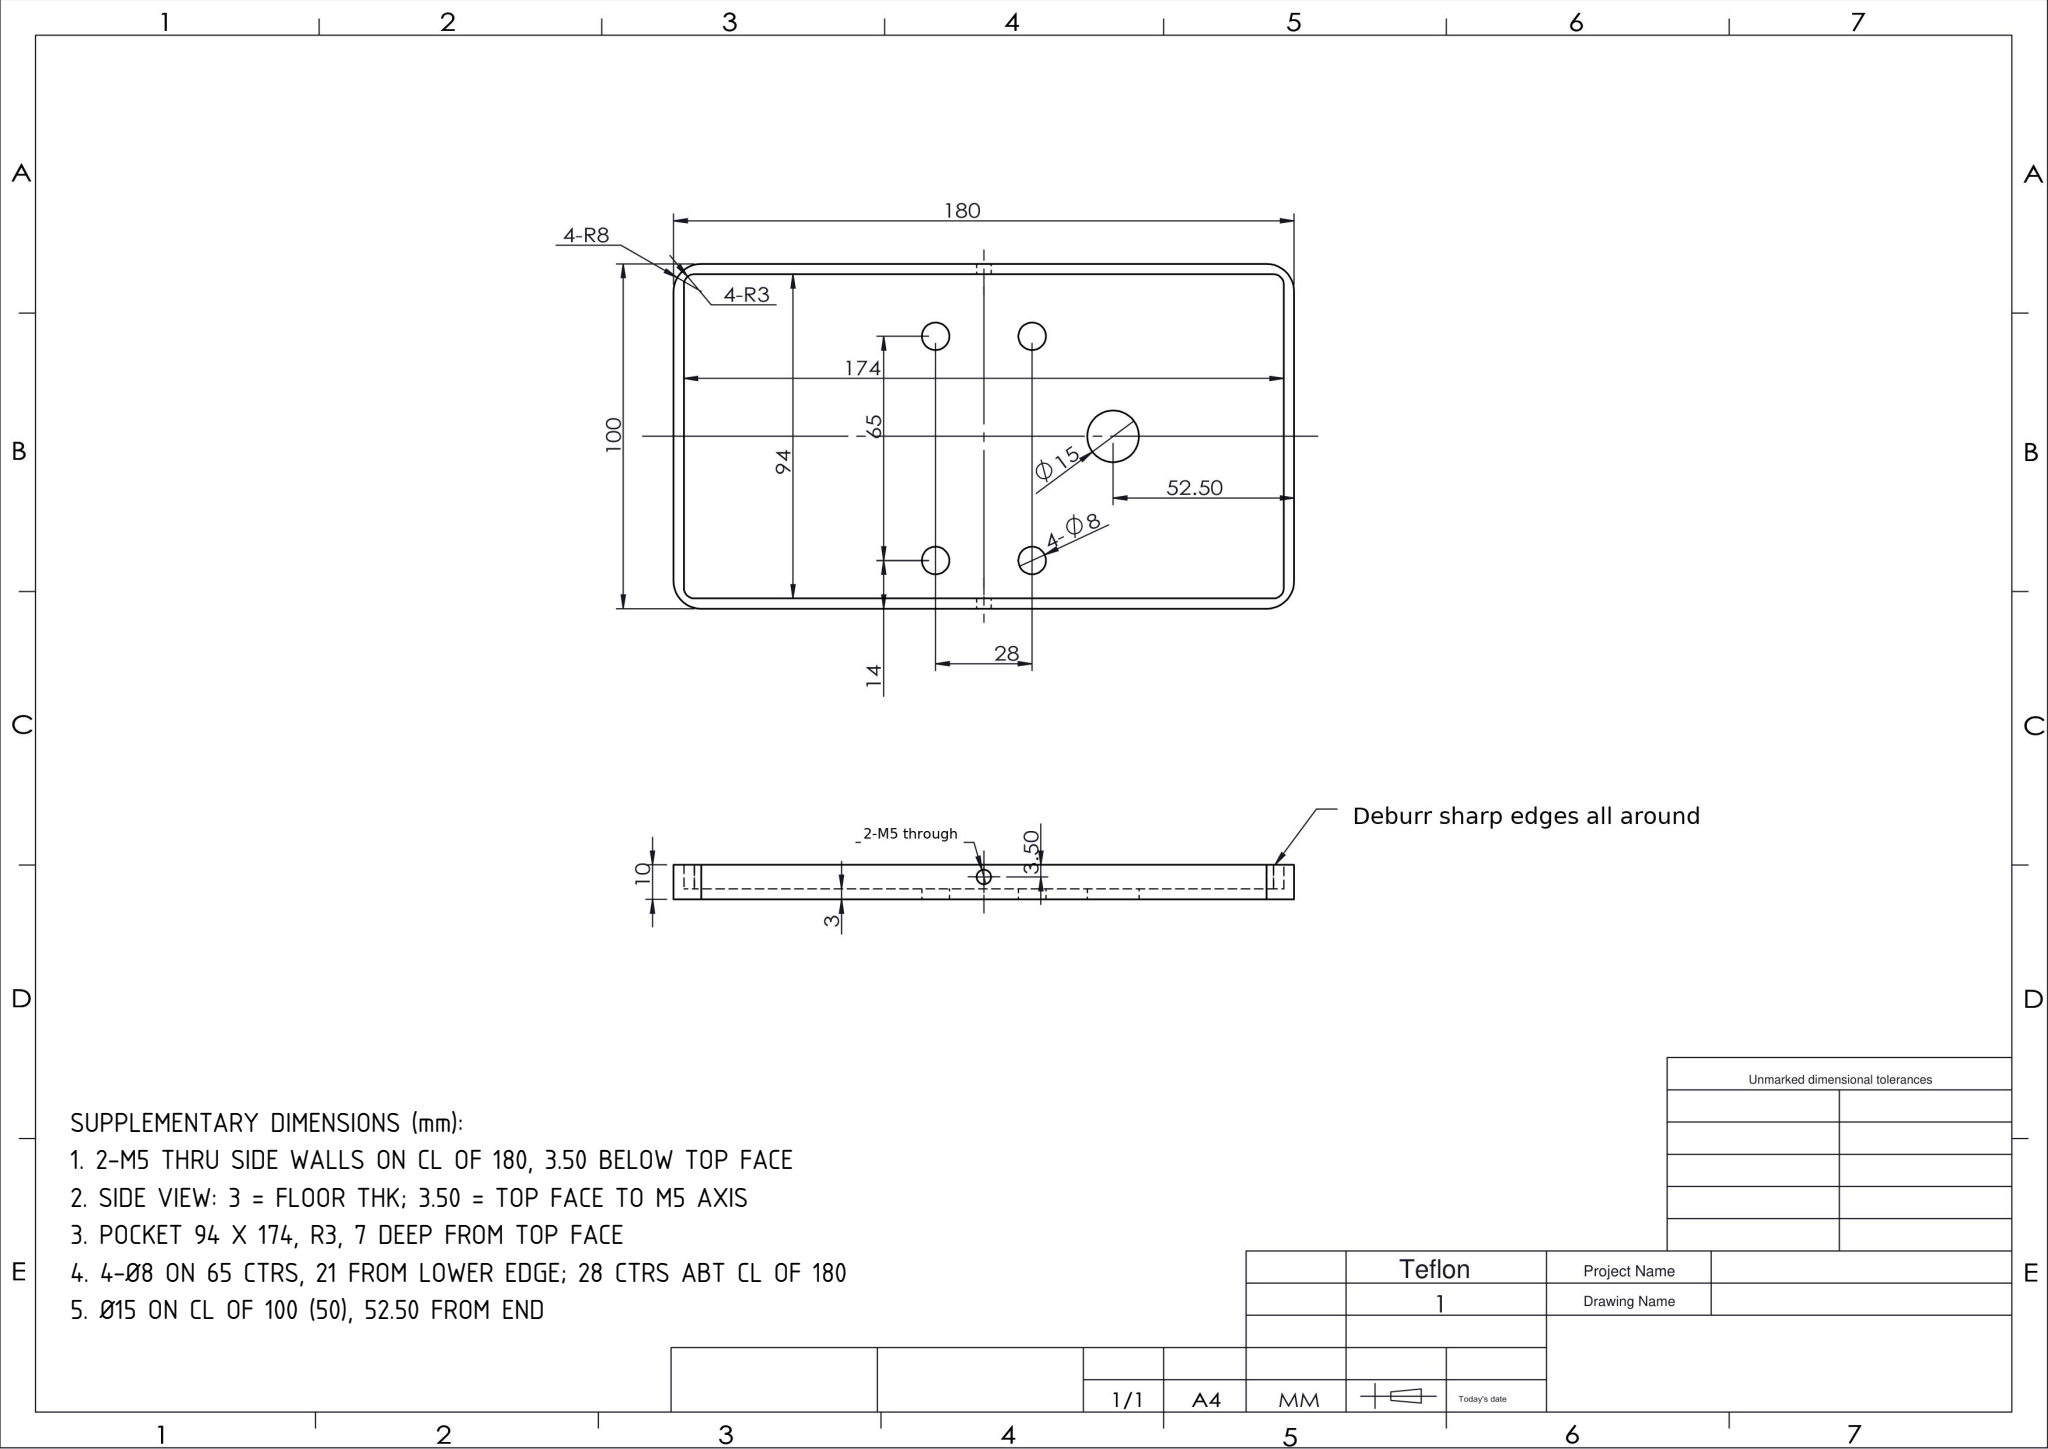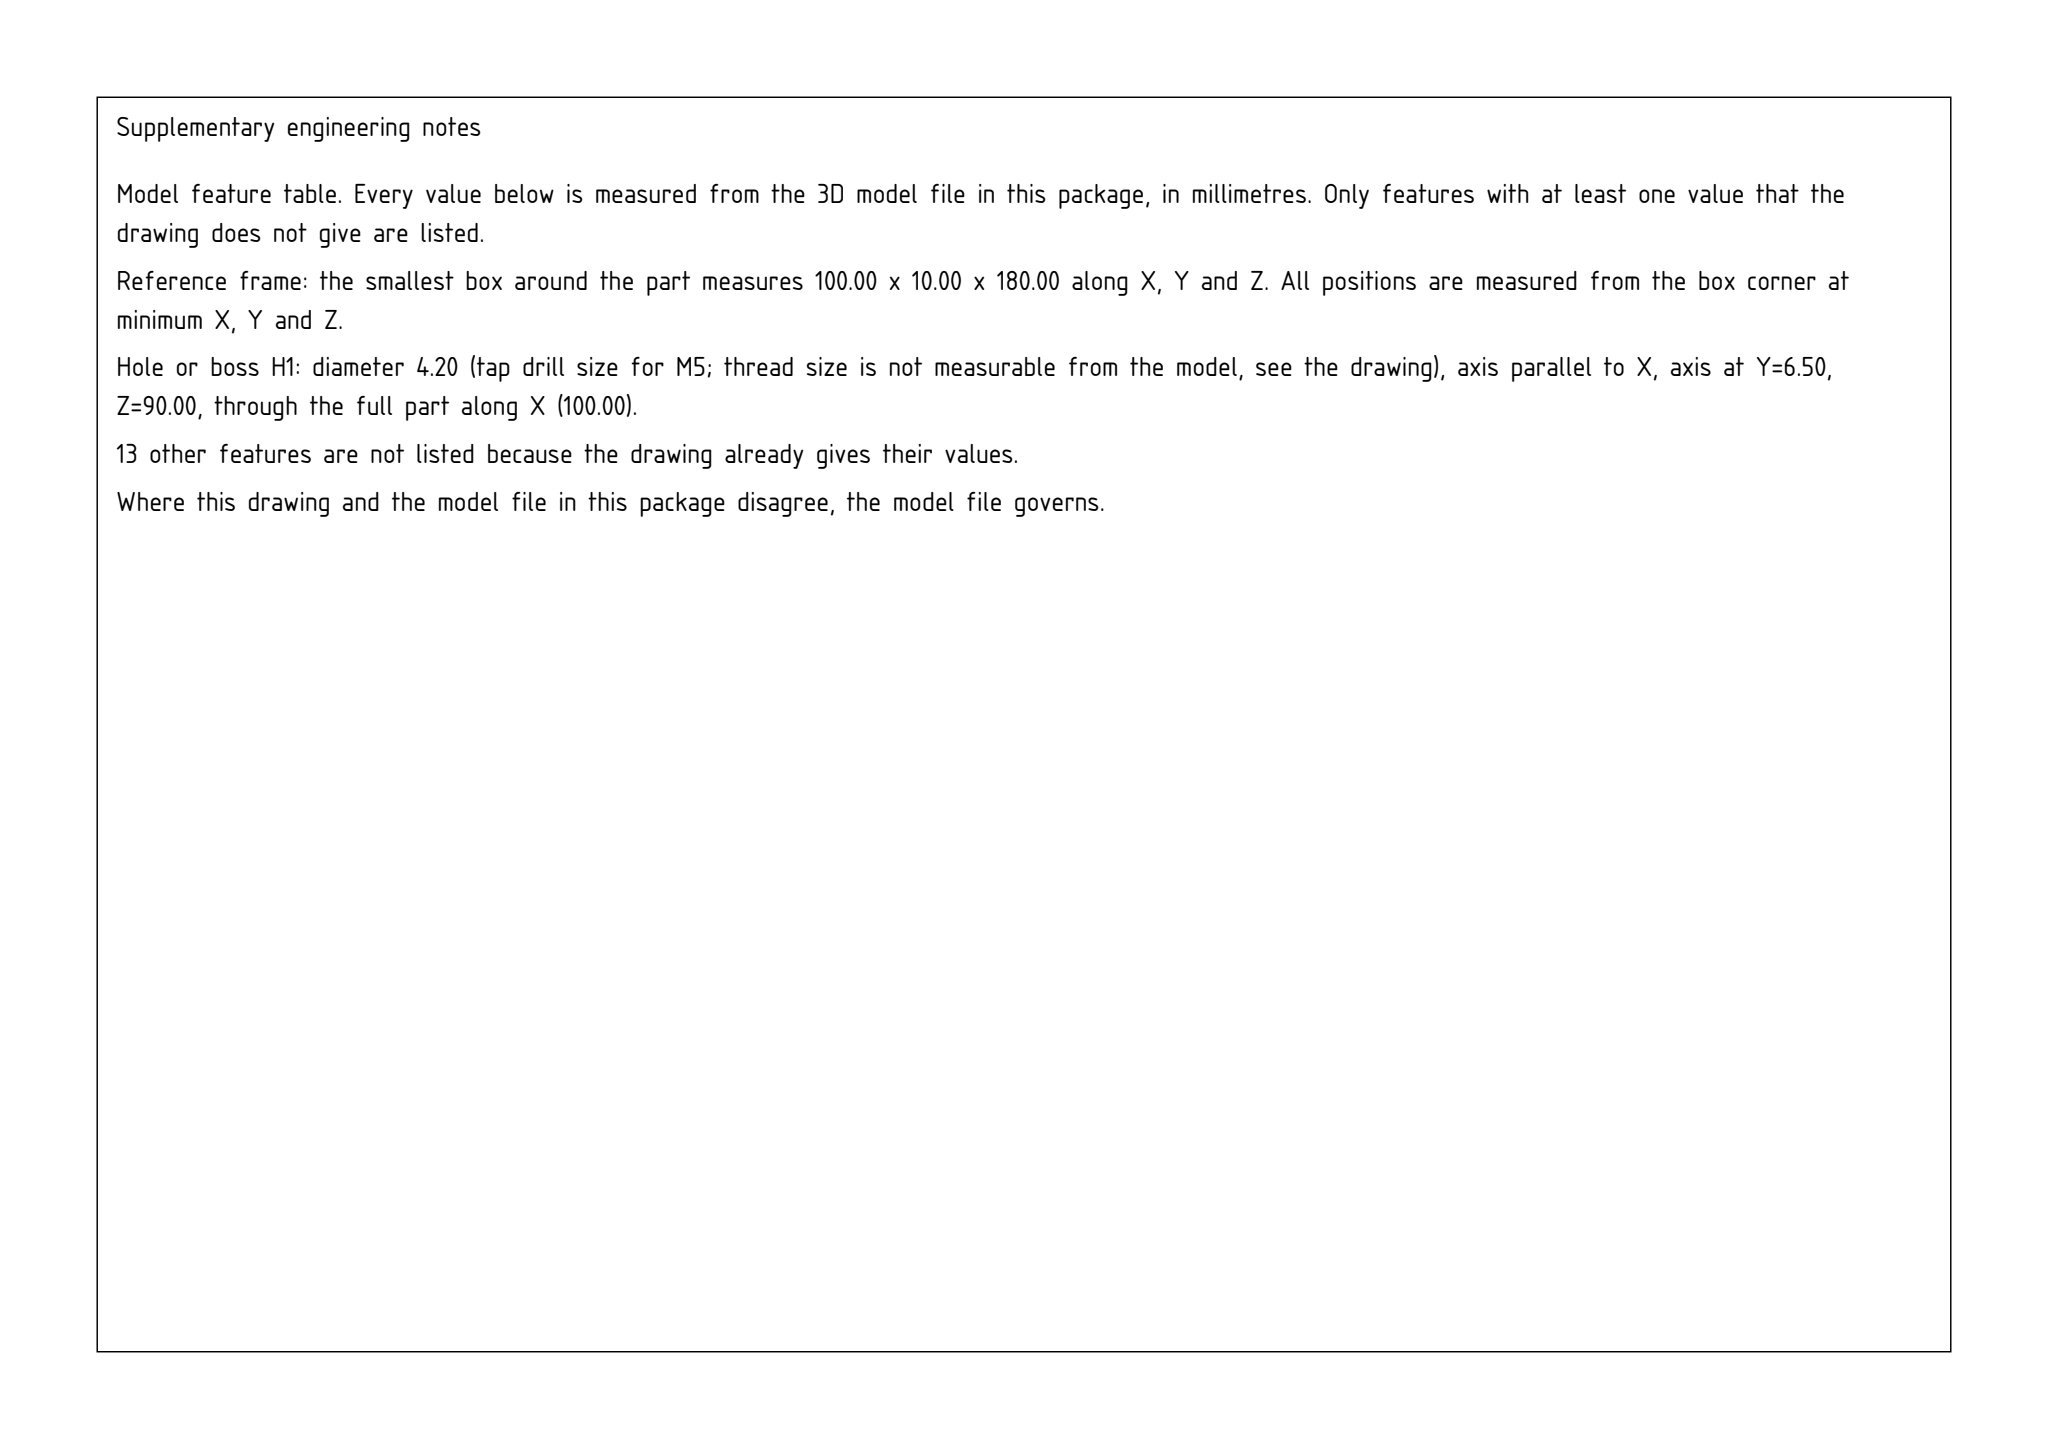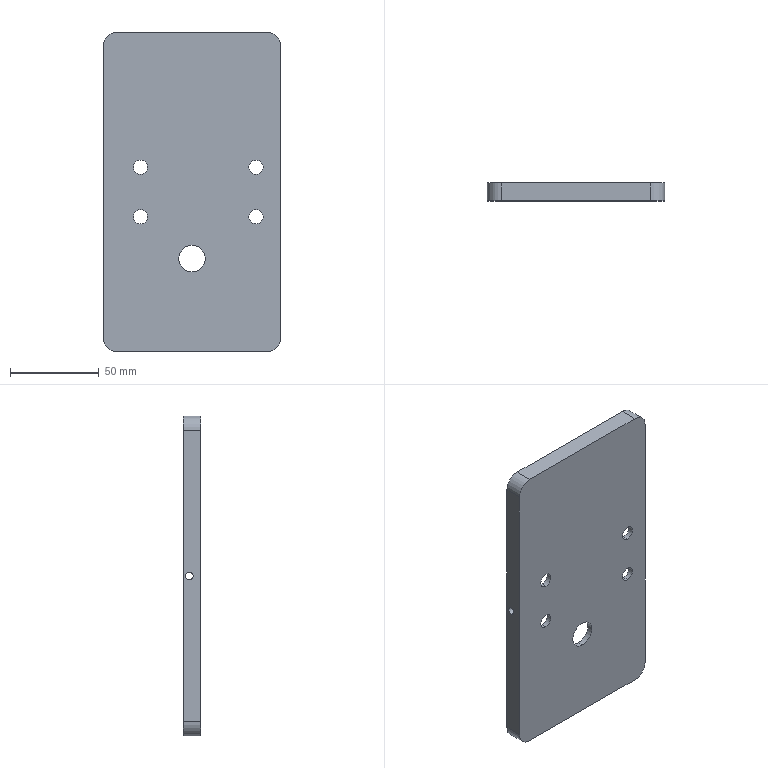Part | SolidWorks | mm | 1 solid | 33 faces | box 100 x 10 x 180 mm | volume 63796 mm3 | cylinder 22 | plane 11 | commonest cylinder face diameters 8 x8 4.2 x4 6 x4 16 x4 15 x2
build123d program:
from build123d import *

# Parameters (mm, degrees)
SKETCH1_W           = 100
SKETCH1_H           = 10
BOSS_EXTRUDE1_DEPTH = 180
SHELL1_T            = -3
M5_TAPPED_HOLE1_D   = 4.2
SKETCH5_R           = 7.5
CUT_EXTRUDE1_DEPTH  = 207.032
FILLET1_R           = 3
FILLET2_R           = 8
SKETCH6_R           = 4
CUT_EXTRUDE2_DEPTH  = 207.032


with BuildPart() as part:
    # Sketch1 → Boss-Extrude1 (new body)
    with BuildSketch(Plane.XY):
        with Locations((50, 5)):
            Rectangle(SKETCH1_W, SKETCH1_H)
    extrude(amount=BOSS_EXTRUDE1_DEPTH)

    # Shell1
    shell1_openings = [part.faces().sort_by_distance(p)[0] for p in [
        (50, 10, 90),
    ]]
    offset(amount=SHELL1_T, openings=shell1_openings, kind=Kind.INTERSECTION)

    # M5 Tapped Hole1 (through all)
    with Locations(Plane(origin=(100, 0, 0), x_dir=(0, 0, -1), z_dir=(1, 0, 0))):
        with Locations((-90, 6.5)):
            Hole(M5_TAPPED_HOLE1_D / 2)

    # Sketch5 → Cut-Extrude1 (cut, through all)
    with BuildSketch(Plane(origin=(0, 3, 0), x_dir=(1, 0, 0), z_dir=(0, 1, 0))):
        with Locations(Location((50, -52.5, 0), (0, 0, 270))):
            Circle(SKETCH5_R)
    extrude(amount=-CUT_EXTRUDE1_DEPTH, mode=Mode.SUBTRACT)

    # Fillet1
    fillet1_edges = [part.edges().sort_by_distance(p)[0] for p in [
        (3, 6.5, 3),
        (97, 6.5, 3),
        (3, 6.5, 177),
        (97, 6.5, 177),
    ]]
    fillet(fillet1_edges, radius=FILLET1_R)

    # Fillet2
    fillet2_edges = [part.edges().sort_by_distance(p)[0] for p in [
        (100, 5, 180),
        (0, 5, 180),
        (100, 5, 0),
        (0, 5, 0),
    ]]
    fillet(fillet2_edges, radius=FILLET2_R)

    # Sketch6 → Cut-Extrude2 (cut, through all)
    with BuildSketch(Plane(origin=(0, 3, 0), x_dir=(1, 0, 0), z_dir=(0, 1, 0))):
        with Locations(Location((86, -76, 0), (0, 0, 270))):
            Circle(SKETCH6_R)
        with Locations(Location((86, -104, 0), (0, 0, 270))):
            Circle(SKETCH6_R)
        with Locations(Location((21, -76, 0), (0, 0, 270))):
            Circle(SKETCH6_R)
        with Locations(Location((21, -104, 0), (0, 0, 270))):
            Circle(SKETCH6_R)
    extrude(amount=-CUT_EXTRUDE2_DEPTH, mode=Mode.SUBTRACT)


solid = part.part